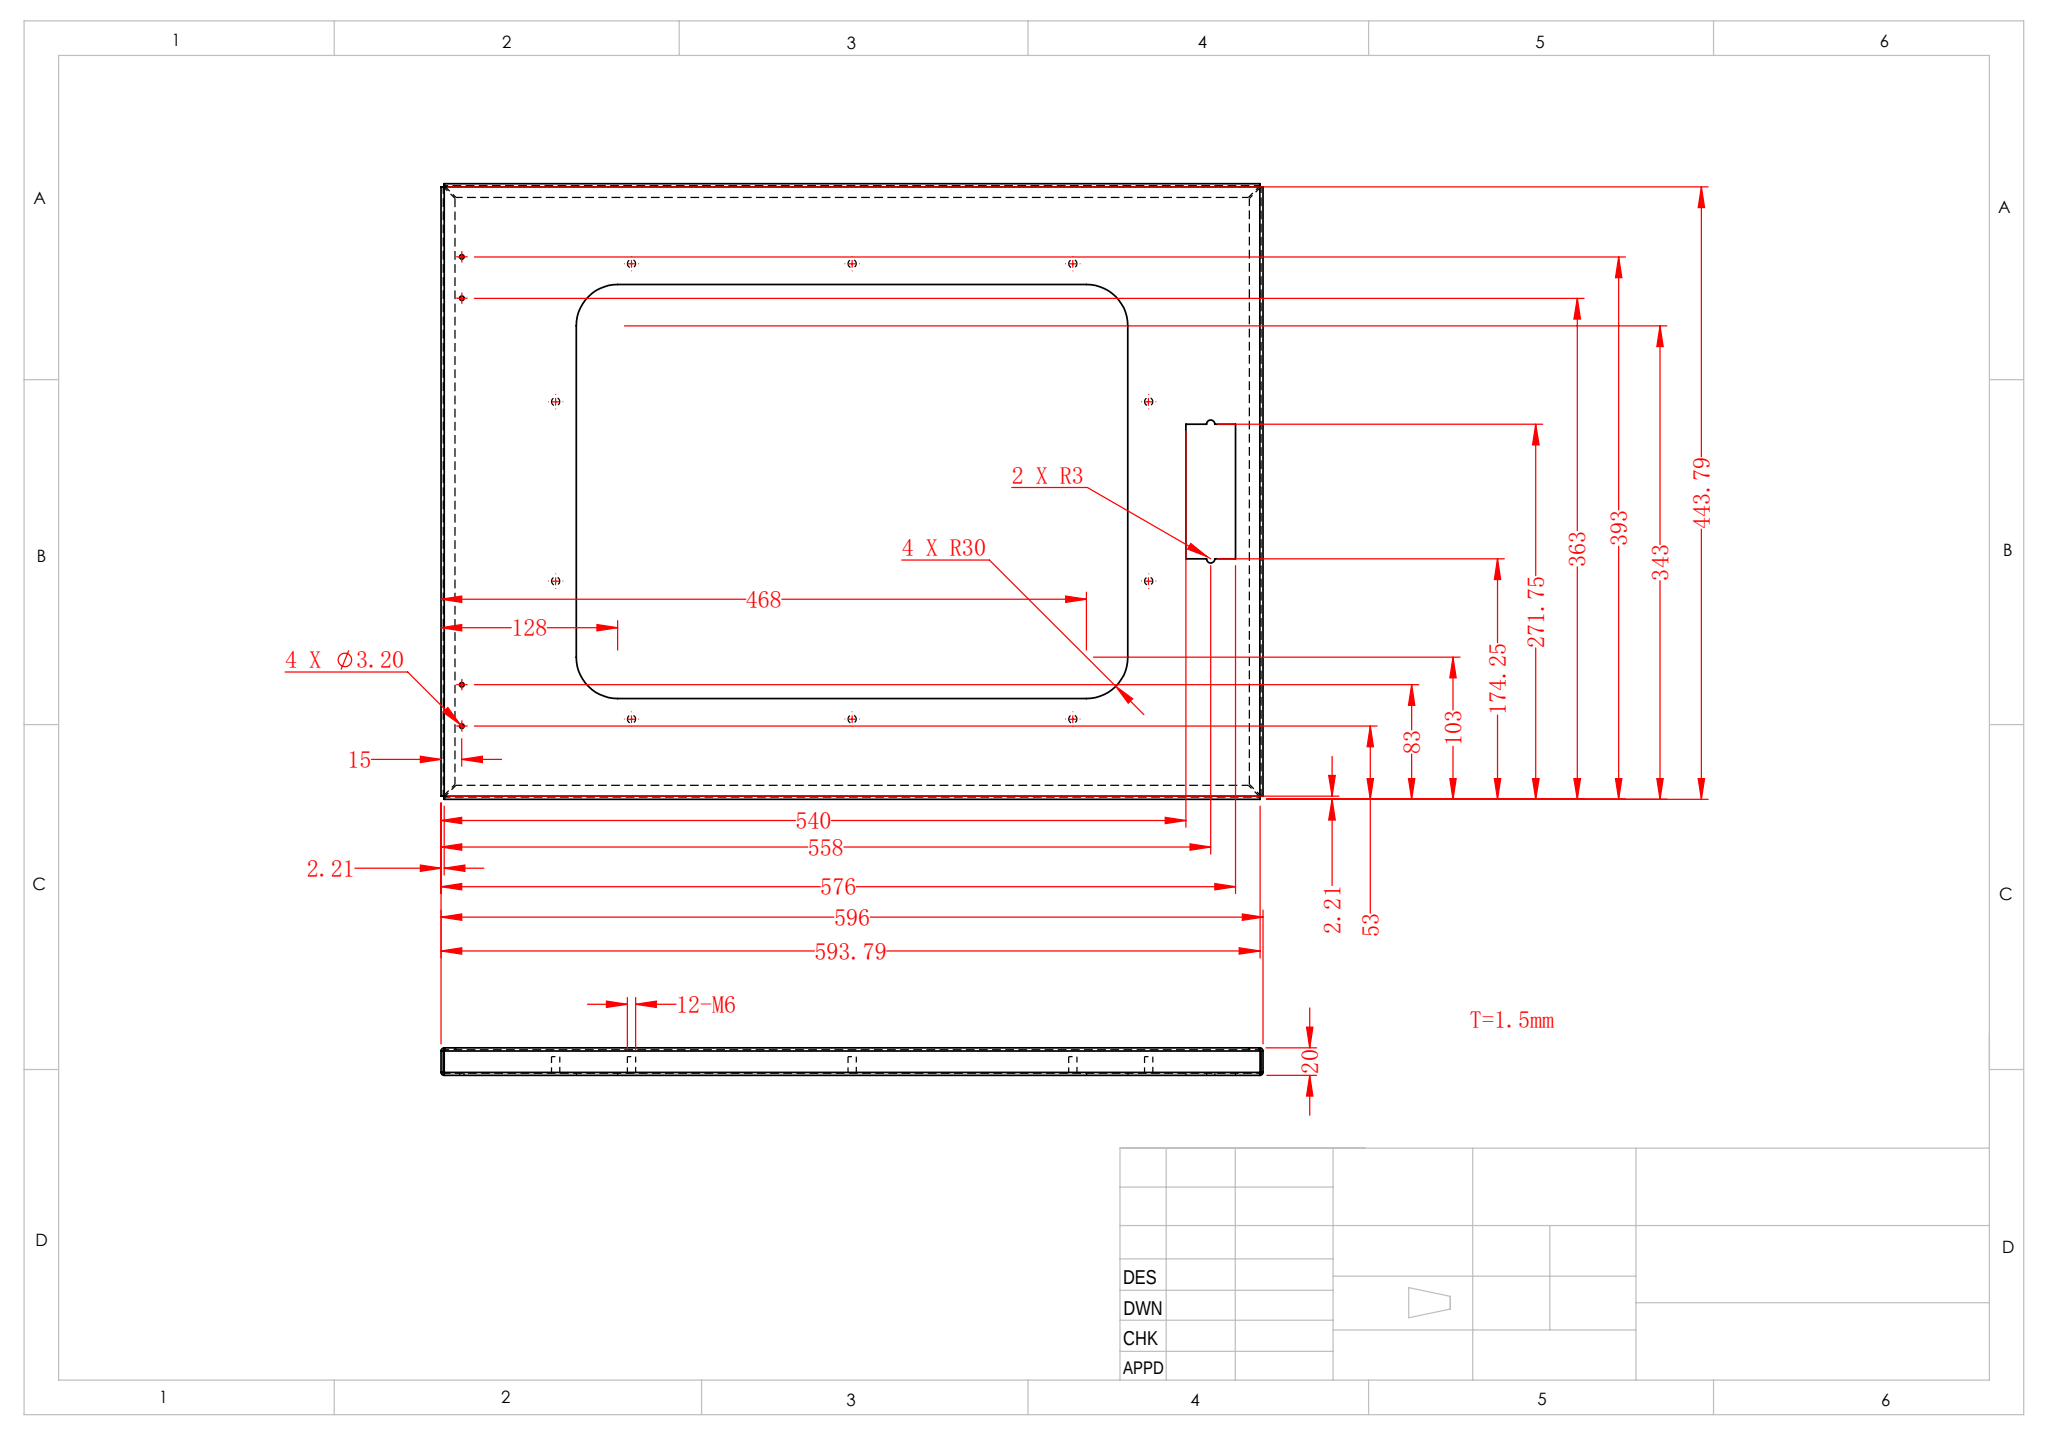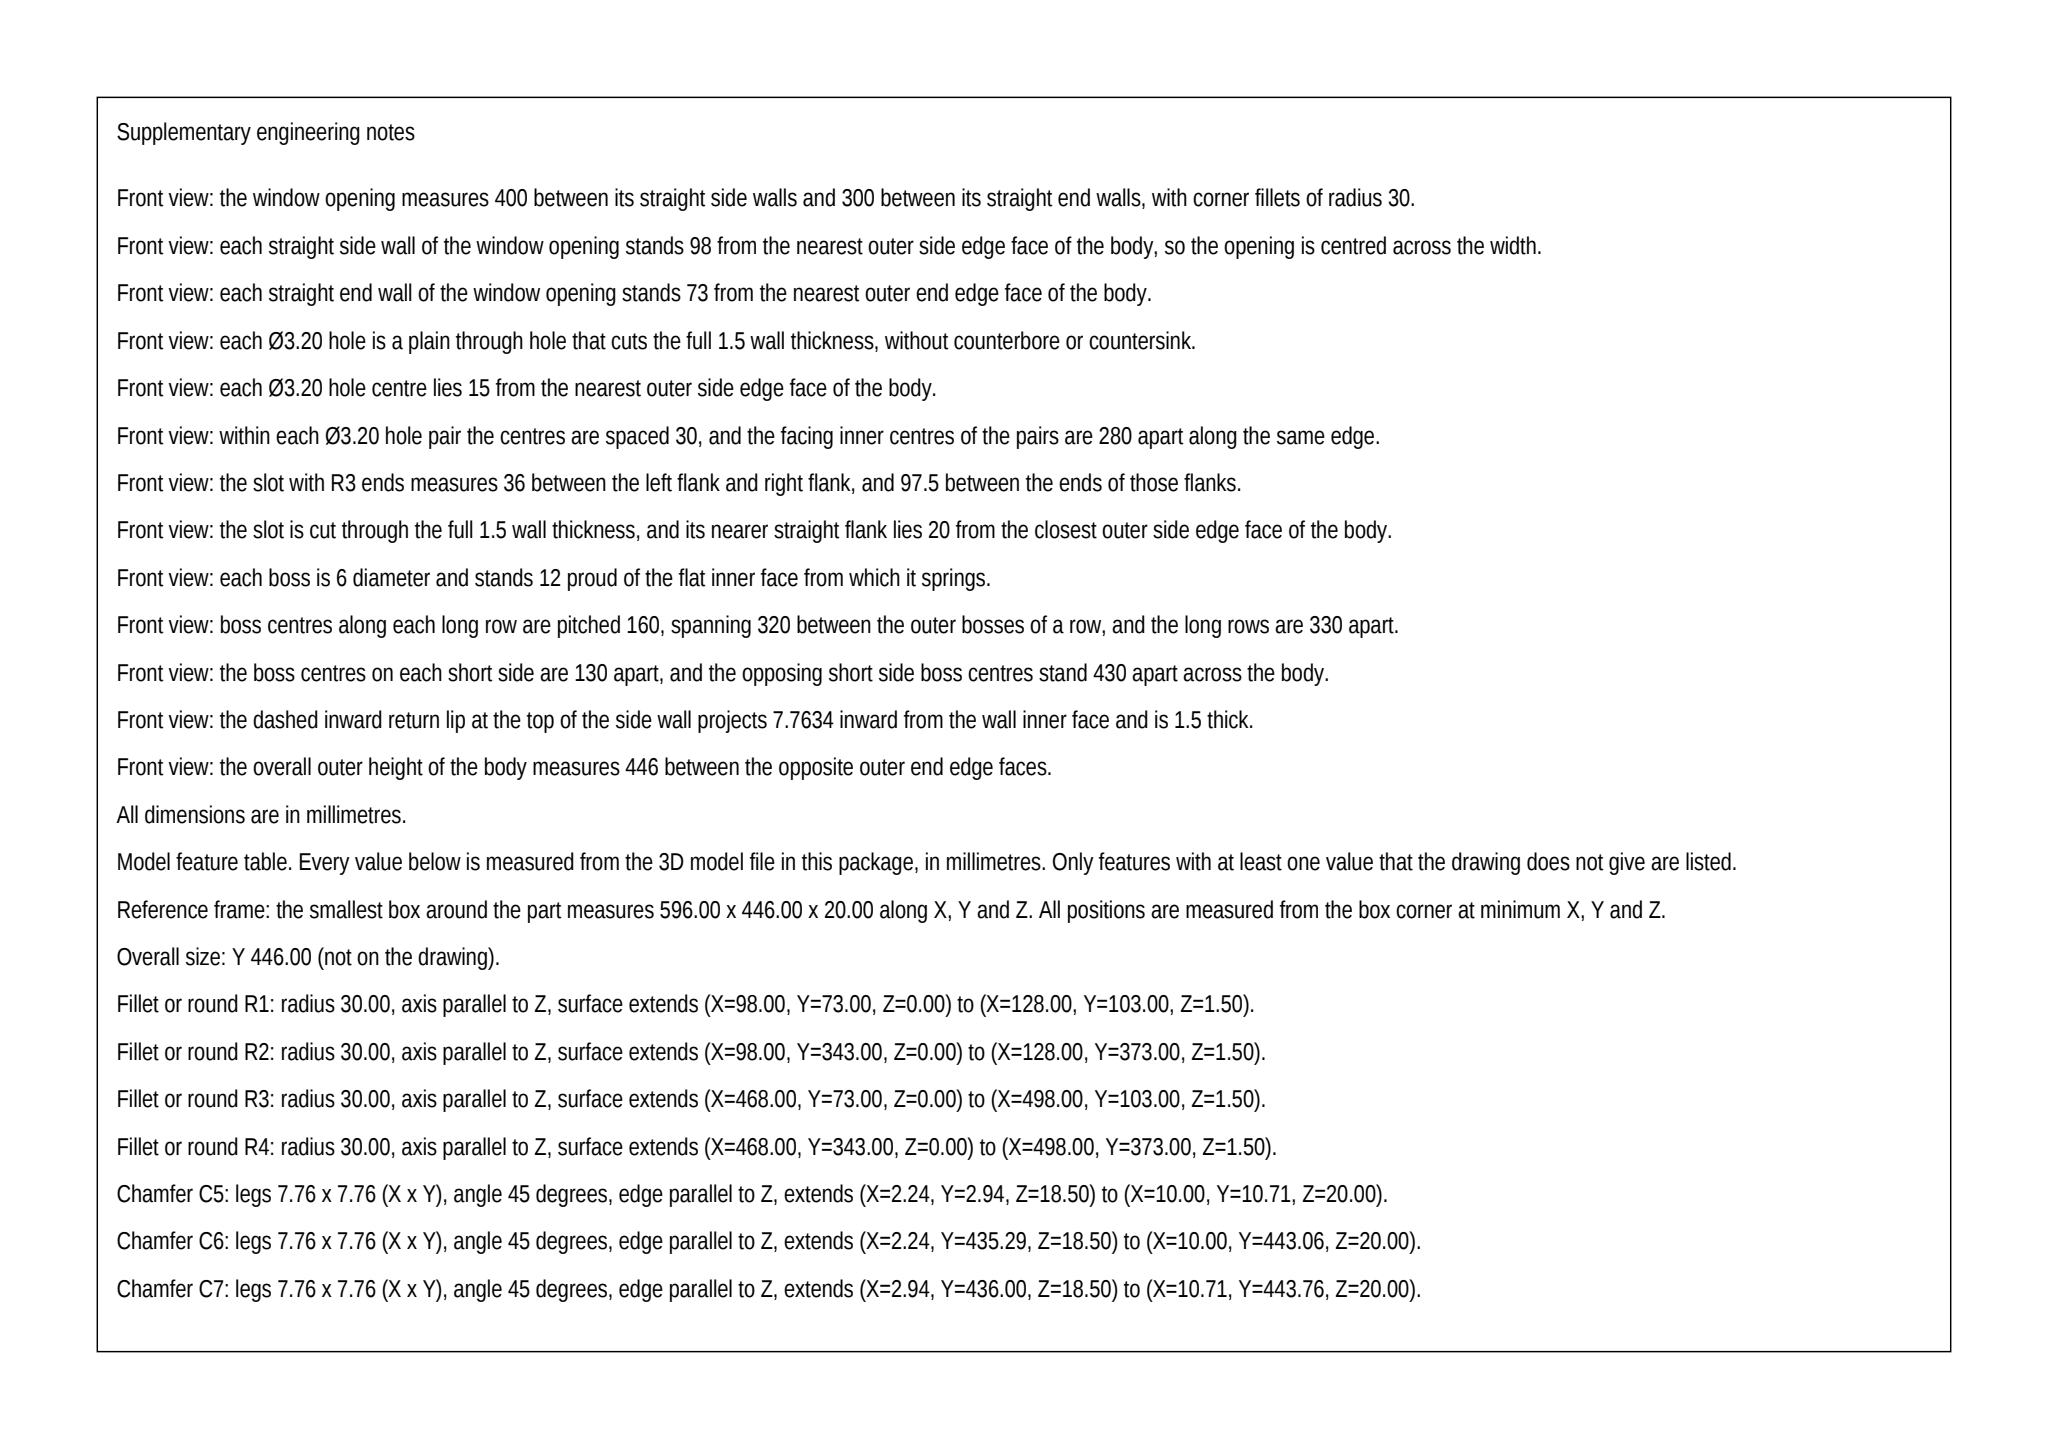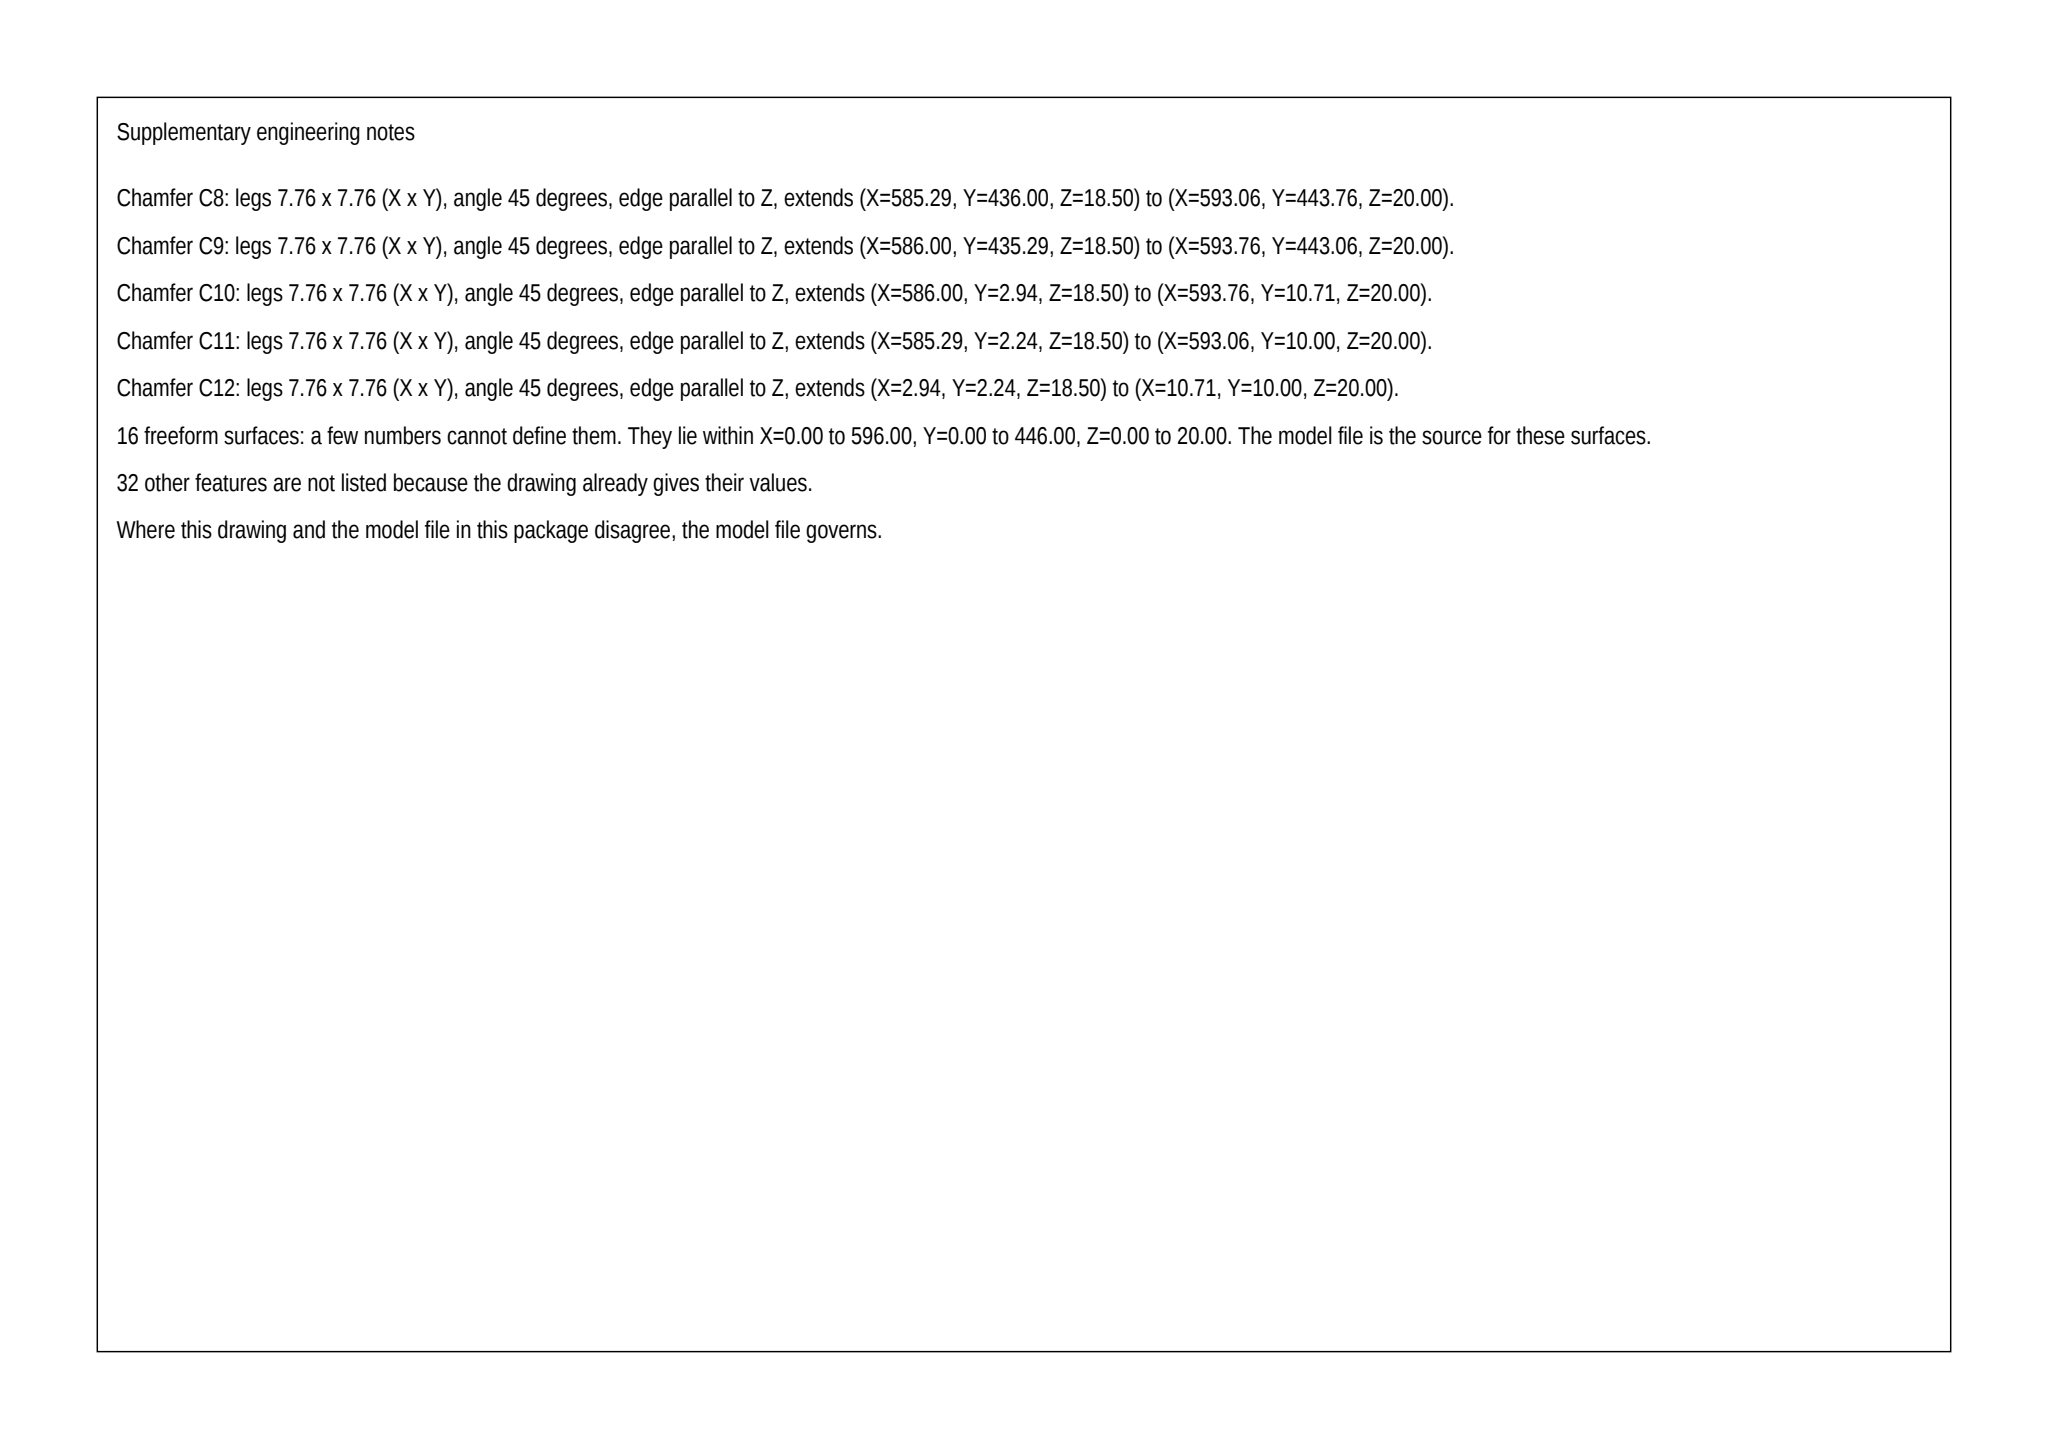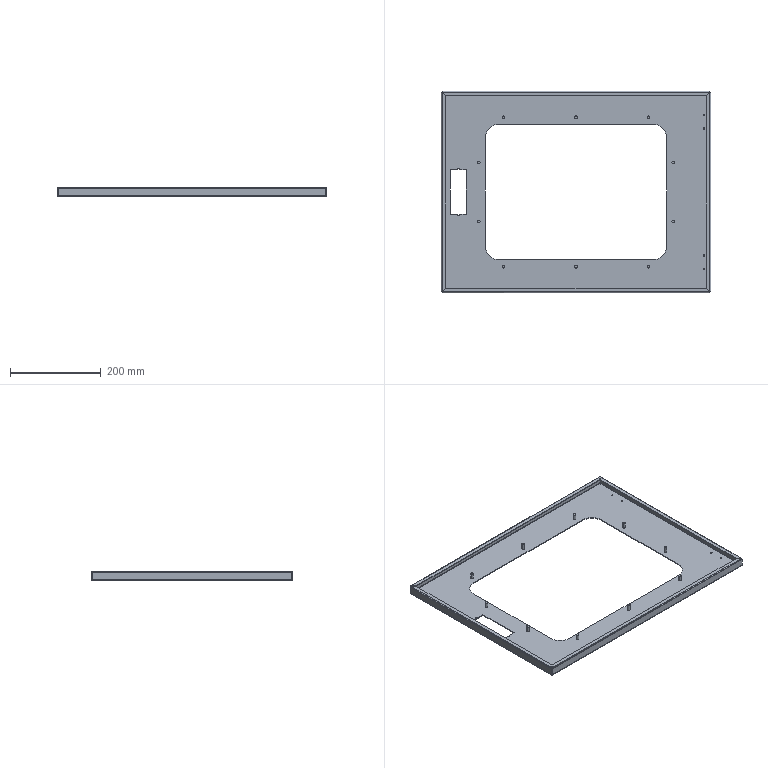Part | SolidWorks | mm | 1 solid | 124 faces | box 596 x 446 x 20 mm | volume 297182 mm3 | plane 58 | cylinder 50 | spline 16 | commonest cylinder face diameters 6 x22 3.2 x8 4.473 x8 1.473 x8 60 x4
Drawing notes:
12-M6 PATTERN LOCATIONS (X,Y from lower-left corner of panel): 10X M6 tapped bosses Ø6.0 x 12 DEEP at (138,58), (298,58), (458,58), (83,158), (513,158), (83,288), (513,288), (138,388), (298,388), (458,388). | from the solid: cylinders dia 6.0, axis z, length 12.0 at [83.02,158.02], [83.02,288.02], [138.02,58.02], [138.02,388.02], [298.02,58.02], [298.02,388.02], [458.02,58.02], [458.02,388.02], [513.02,158.02], [513.02,288.02]
2X Ø6.0 THRU (through 1.5 panel) at X=38 from left edge, Y=174.25 and Y=271.75 from bottom edge. | from the solid: cylinders dia 6.0, axis z, length 1.5 at [38.02,174.27] and [38.02,271.77]
4X Ø3.20 THRU at X=581 from left edge (15 from right edge), Y=53, 83, 363 and 393 from bottom edge. | from the solid: cylinders dia 3.2, axis z, length 1.5 at [581.02,53.02], [581.02,83.02], [581.02,363.02], [581.02,393.02]
ALL FORMED FLANGES (20 HIGH, 4 SIDES): BEND ANGLE 90°, INSIDE BEND RADIUS R0.74, OUTSIDE R2.24, MATERIAL T=1.5. | from the solid: concentric bend cylinders dia 1.473 (R0.737 inside) and dia 4.473 (R2.237 outside) on x and y axes at [2.25,2.25], [2.25,17.78], [443.78,2.25], [443.78,17.78] / [593.78,...]; orthogonal axis_planes z 0.02/20.02 give 90° bend; bbox z = 20.03
UNSPECIFIED BEND RADII: R0.74 INSIDE (all bends per model). | from the solid: fillet_radii list empty; only bend cylinders dia 1.473 / 4.473 present in model
INWARD RETURN LIP (HEM) AT TOP OF ALL FOUR 20 HIGH FLANGES: LIP LEG 8.5 WIDE MEASURED FROM INSIDE FACE OF FLANGE (INNER EDGE 10.0 FROM OUTSIDE FACE OF FLANGE, i.e. X=10.0 AND X=586.0 FROM LEFT EDGE, Y=10.0 AND Y=436.0 FROM BOTTOM EDGE). | from the solid: axis_planes x=10.02 and 586.02, y=10.02 and 436.02 (lip inner edges) vs inner flange faces x=1.52/594.52 and y=1.52/444.52; bbox 596.03 x 446.03
RETURN LIP MATERIAL THICKNESS 1.5, LIP TOP FACE FLUSH WITH TOP OF FLANGE AT 20.0 ABOVE PANEL OUTSIDE FACE; LIP UNDERSIDE AT 18.5 ABOVE PANEL OUTSIDE FACE. | from the solid: axis_planes z=18.52 (4) and z=20.02 (4) with z=0.02 panel outside face; bbox Z=20.03